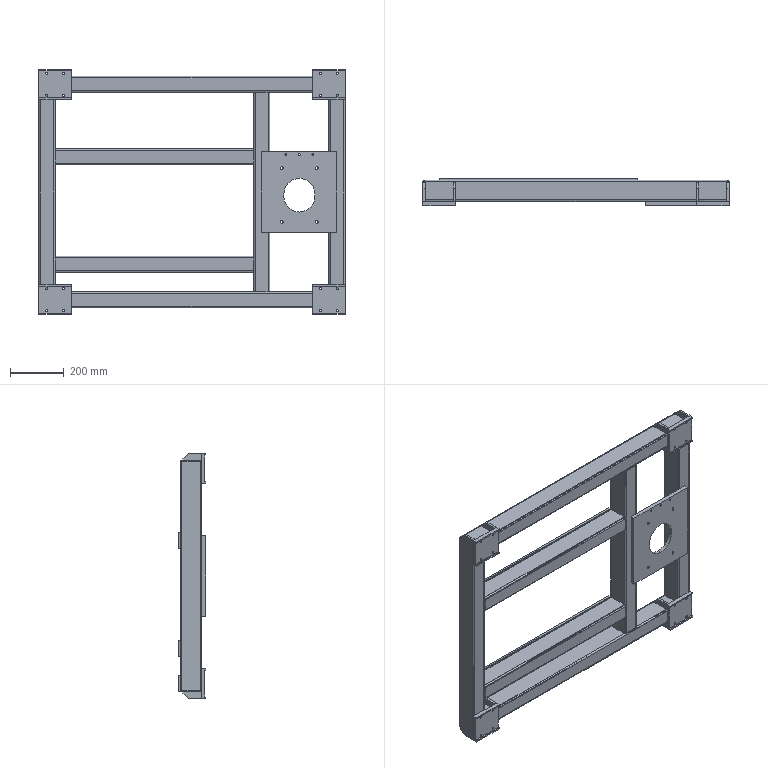Component | SolidWorks | SupportFrame1-1 | 27 solids | 392 faces | volume 7106095 mm3 | plane 225 | cylinder 167 | commonest cylinder face diameters 8.5 x40 6.8 x40 12 x28 6 x28 5 x16 10.2 x8 10 x4 115 x3